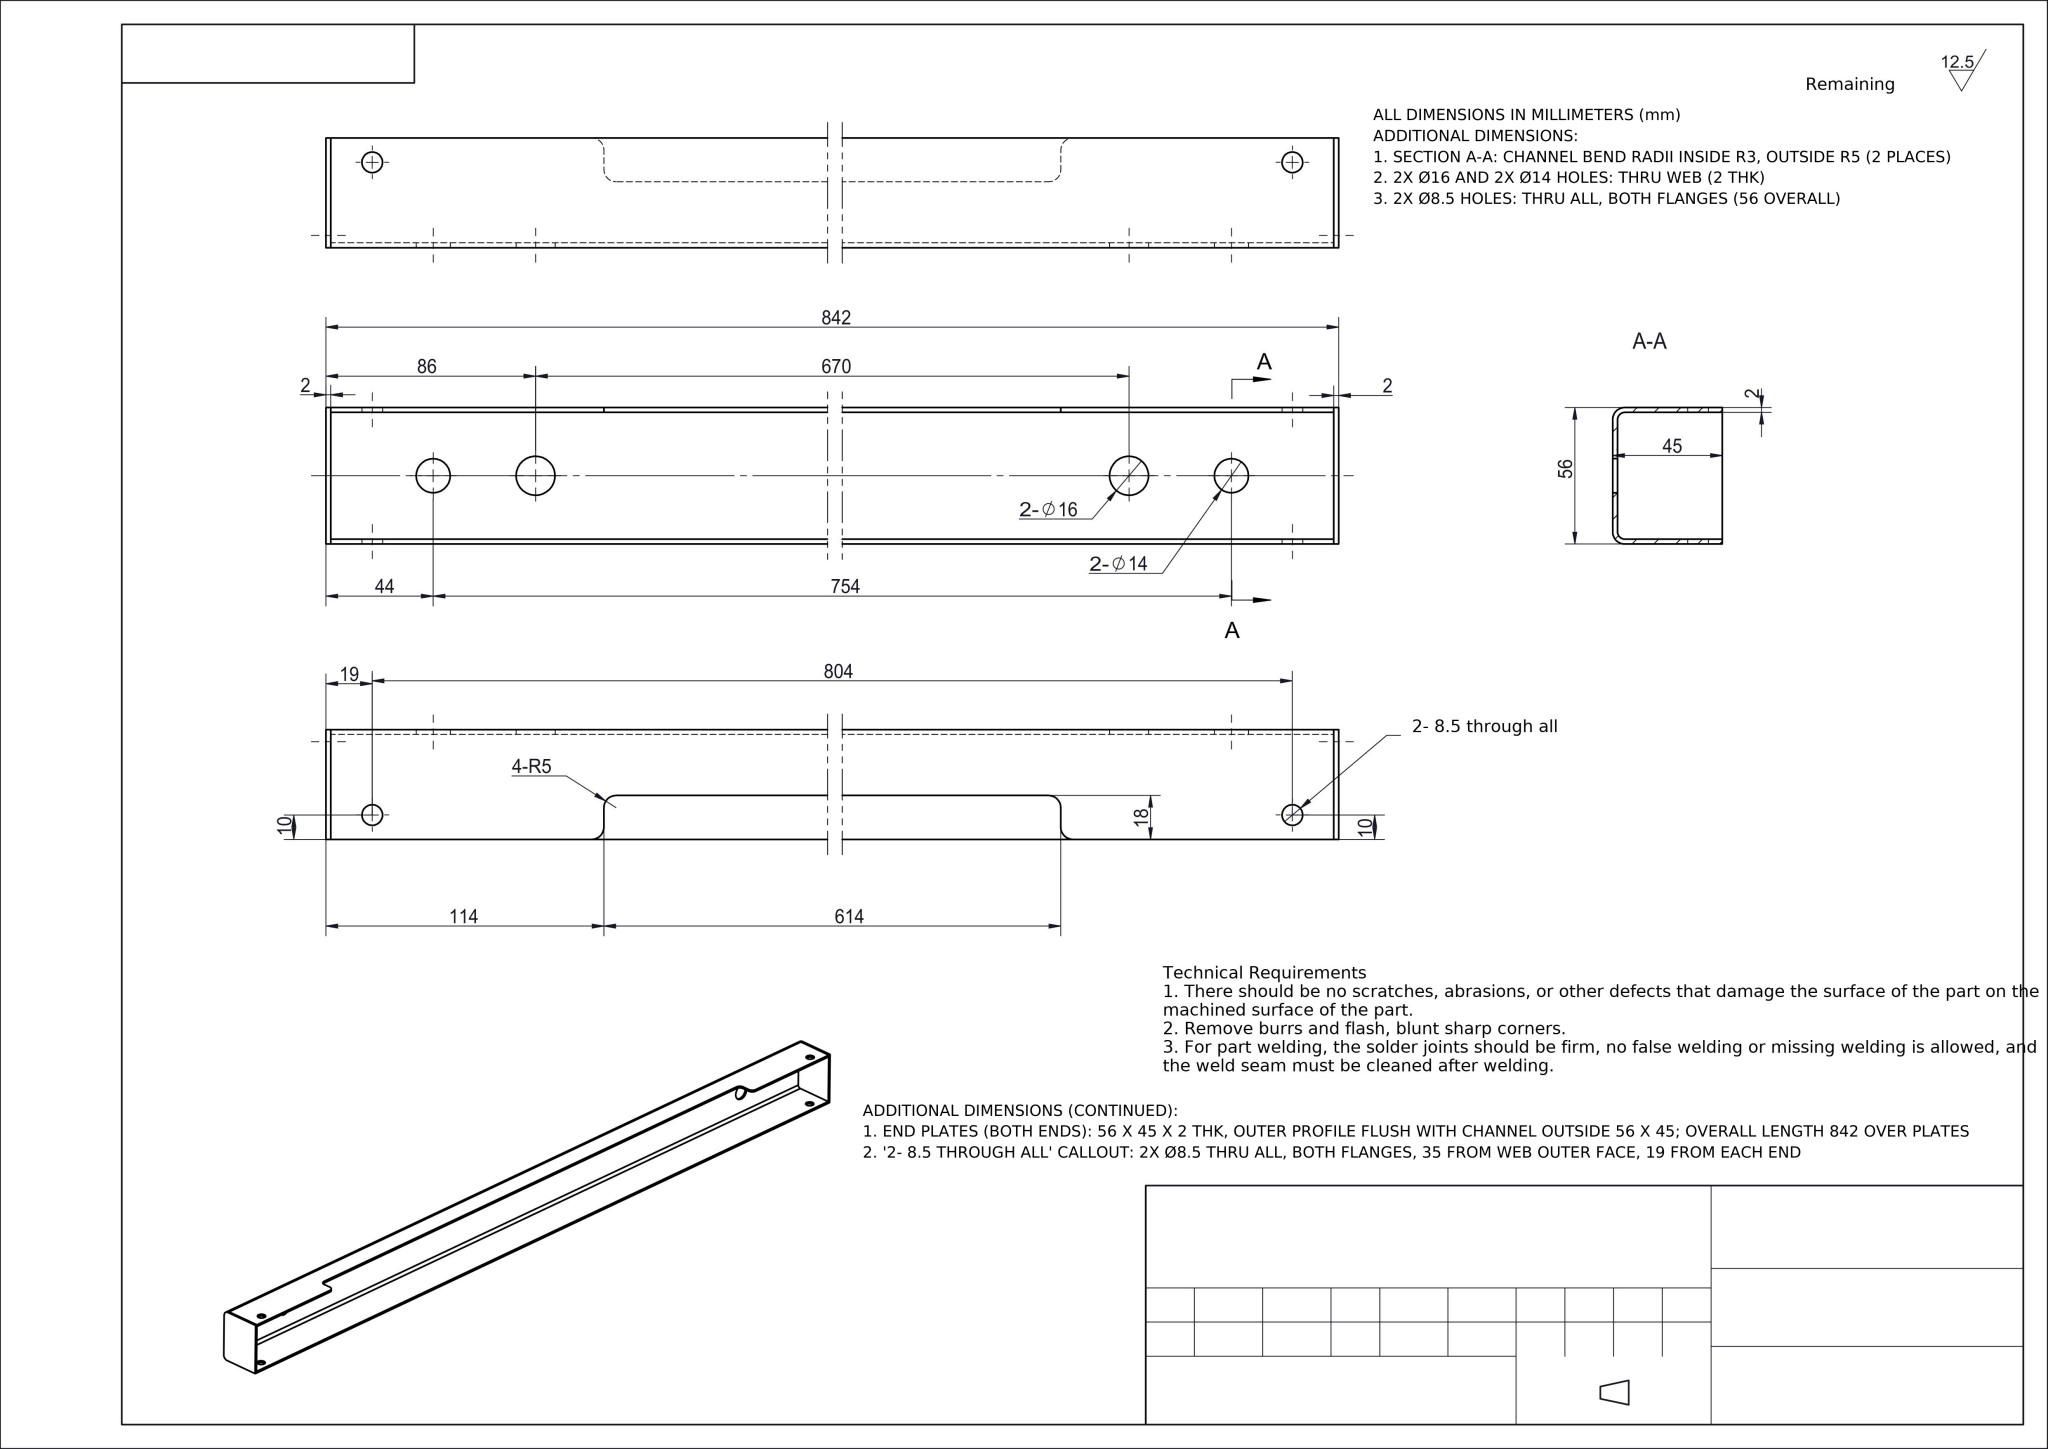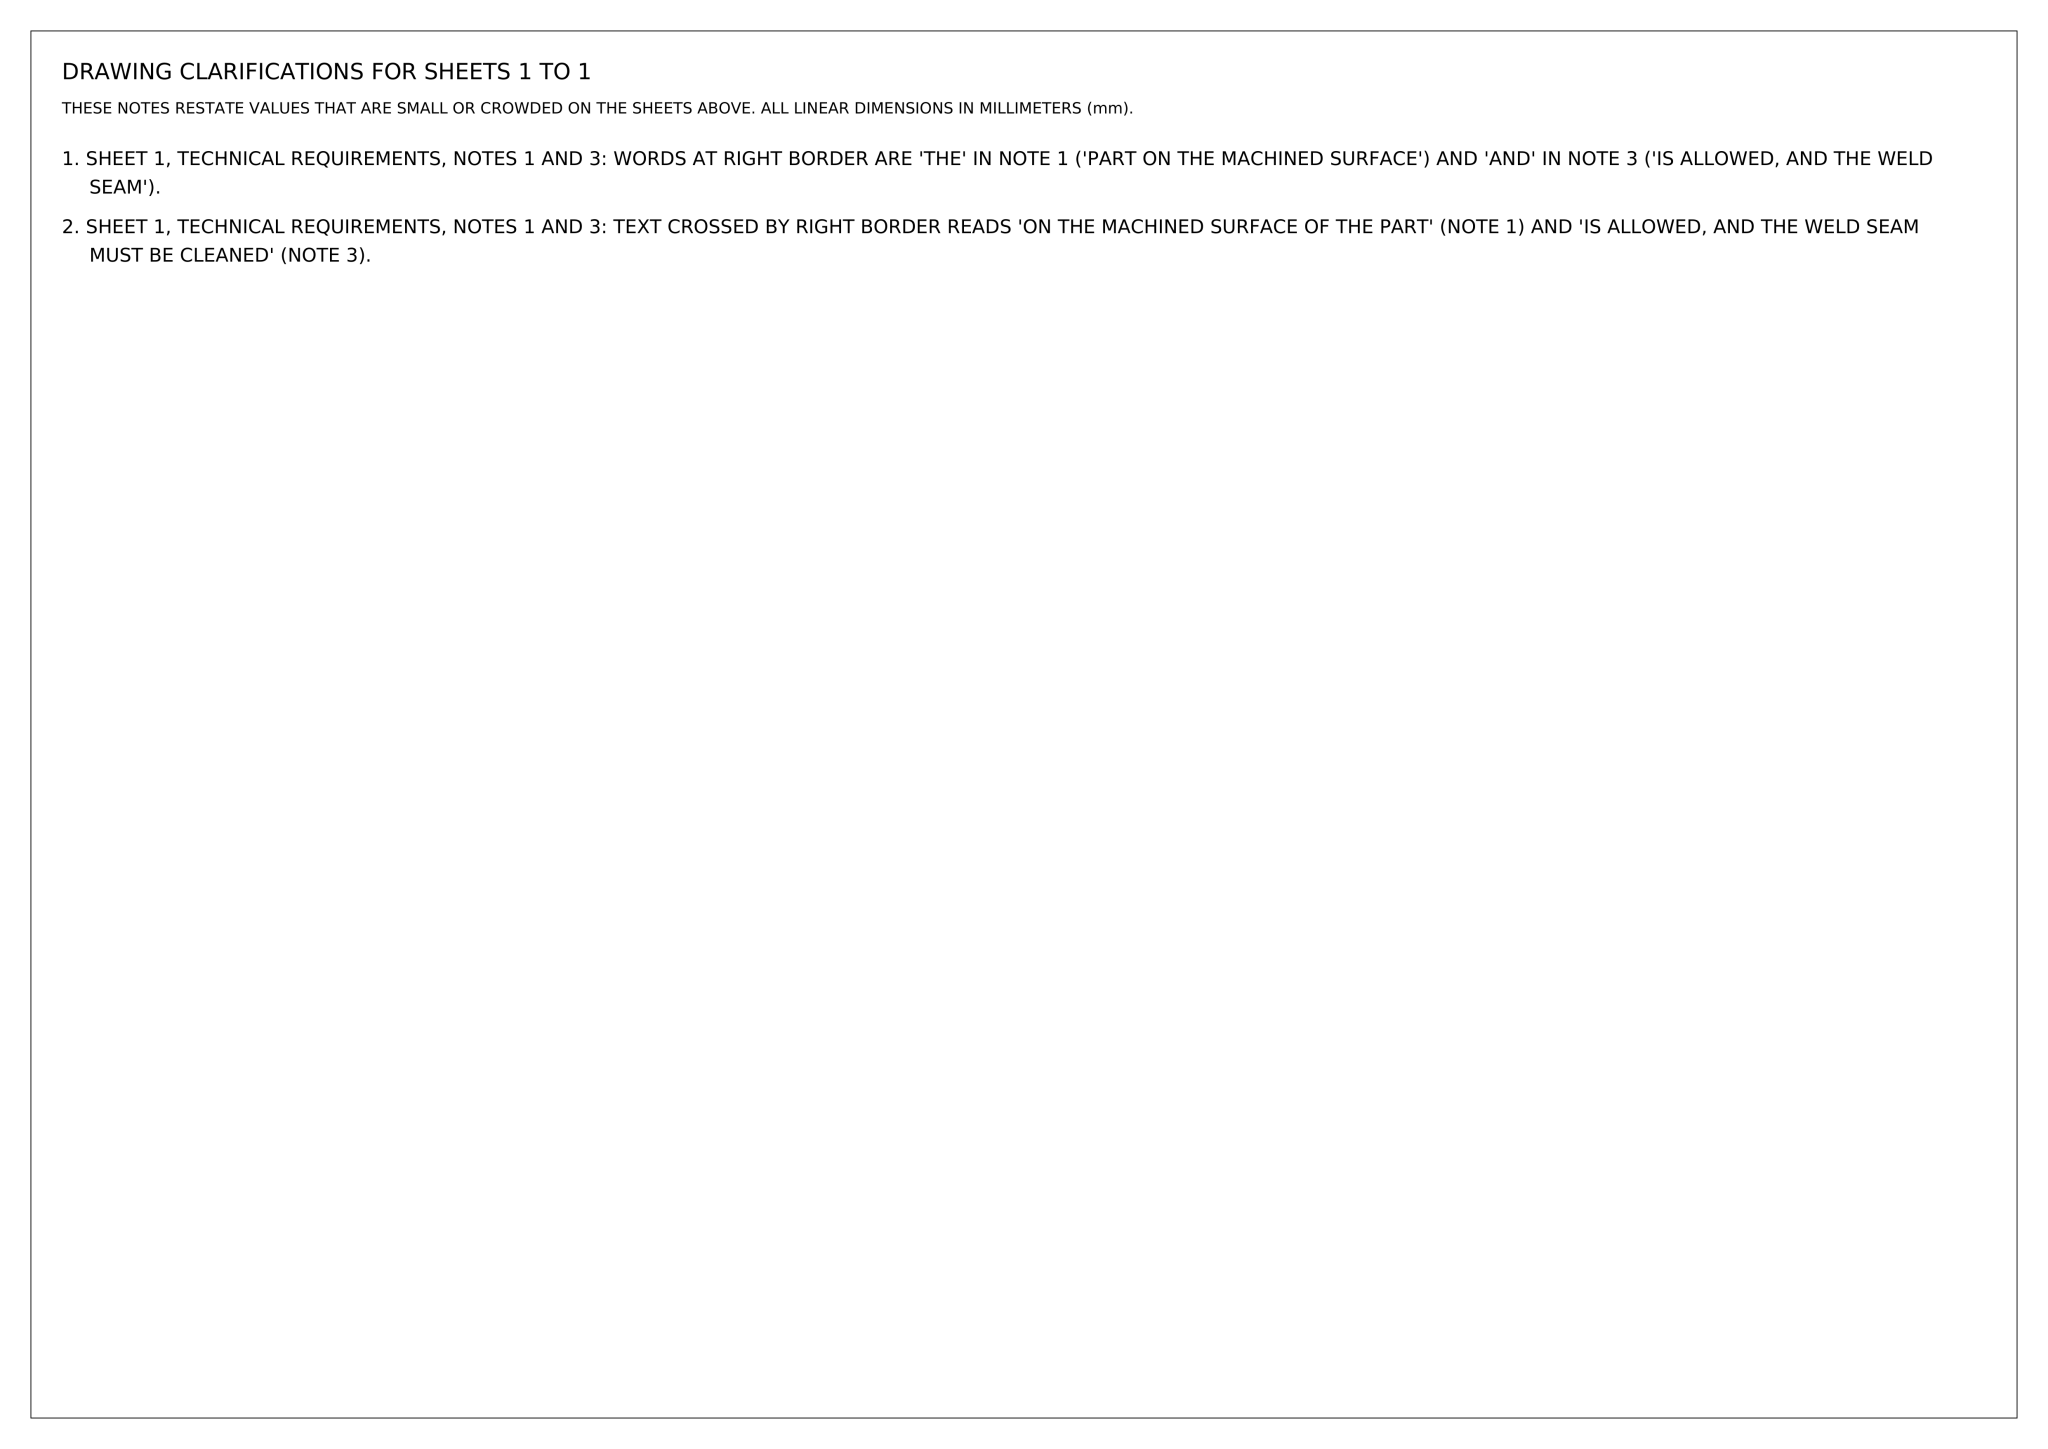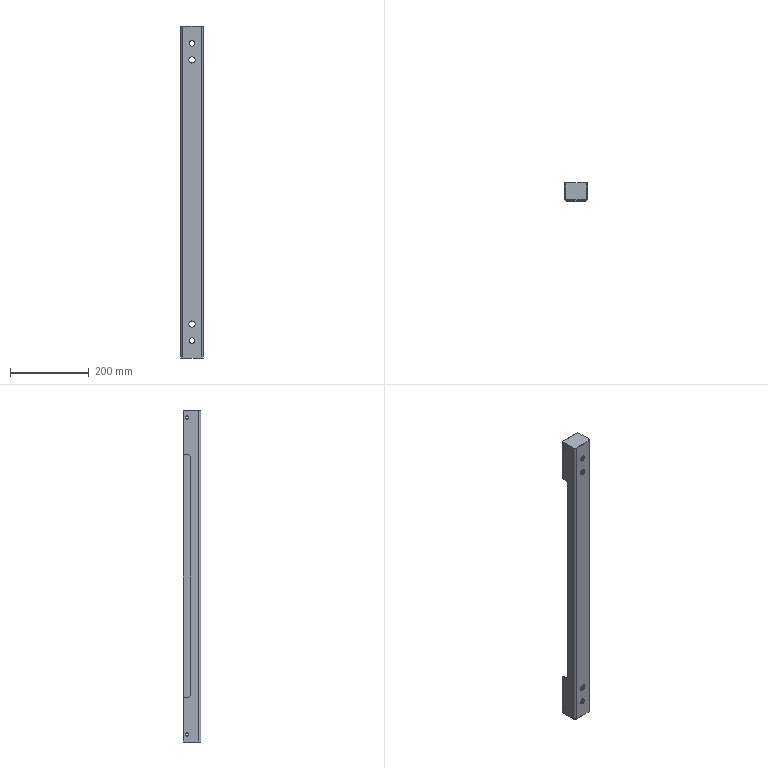Part | NX | mm | 1 solid | 38 faces | box 56 x 45 x 842 mm | volume 218296 mm3 | cylinder 24 | plane 14 | commonest cylinder face diameters 8.5 x8 10 x6 16 x4 14 x4 6 x2